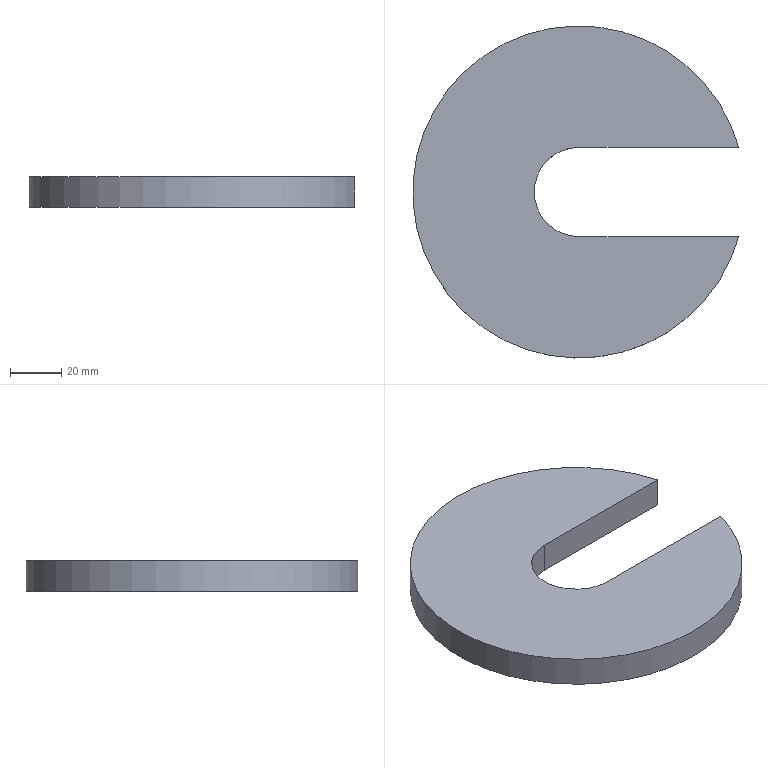Component | NX | QC_WASHER | 1 solid | 6 faces | box 127.6 x 130 x 12 mm | volume 126540 mm3 | plane 4 | cylinder 2 | commonest cylinder face diameters 35 x1 130 x1
STEP:
#1=CARTESIAN_POINT('',(0.,0.,0.));
#2=DIRECTION('',(0.,0.,1.));
#3=DIRECTION('',(1.,0.,0.));
#4=AXIS2_PLACEMENT_3D('',#1,#2,#3);
#5=CARTESIAN_POINT('',(62.6,-17.5,123.));
#6=VERTEX_POINT('',#5);
#7=CARTESIAN_POINT('',(0.,-17.5,123.));
#8=VERTEX_POINT('',#7);
#9=CARTESIAN_POINT('',(62.6,-17.5,123.));
#10=DIRECTION('',(-1.,-0.,0.));
#11=VECTOR('',#10,1.);
#12=LINE('',#9,#11);
#13=CARTESIAN_POINT('',(62.6,-17.5,135.));
#14=DIRECTION('',(0.,-1.,0.));
#15=DIRECTION('',(1.,0.,0.));
#16=AXIS2_PLACEMENT_3D('',#13,#14,#15);
#17=PLANE('',#16);
#18=CARTESIAN_POINT('',(0.,-12.));
#19=DIRECTION('',(-1.,0.));
#20=VECTOR('',#19,1.);
#21=LINE('',#18,#20);
#22=(GEOMETRIC_REPRESENTATION_CONTEXT(2)PARAMETRIC_REPRESENTATION_CONTEXT()REPRESENTATION_CONTEXT('',''));
#23=DEFINITIONAL_REPRESENTATION('',(#21),#22);
#24=PCURVE('',#17,#23);
#25=CARTESIAN_POINT('',(0.,0.,123.));
#26=DIRECTION('',(0.,0.,-1.));
#27=DIRECTION('',(0.,-1.,0.));
#28=AXIS2_PLACEMENT_3D('',#25,#26,#27);
#29=PLANE('',#28);
#30=CARTESIAN_POINT('',(17.5,-62.6));
#31=DIRECTION('',(0.,1.));
#32=VECTOR('',#31,1.);
#33=LINE('',#30,#32);
#34=(GEOMETRIC_REPRESENTATION_CONTEXT(2)PARAMETRIC_REPRESENTATION_CONTEXT()REPRESENTATION_CONTEXT('',''));
#35=DEFINITIONAL_REPRESENTATION('',(#33),#34);
#36=PCURVE('',#29,#35);
#37=SURFACE_CURVE('',#12,(#24,#36),.PCURVE_S1.);
#38=EDGE_CURVE('',#6,#8,#37,.T.);
#39=ORIENTED_EDGE('',*,*,#38,.T.);
#40=CARTESIAN_POINT('',(0.,-17.5,135.));
#41=VERTEX_POINT('',#40);
#42=CARTESIAN_POINT('',(0.,-17.5,135.));
#43=DIRECTION('',(0.,0.,-1.));
#44=VECTOR('',#43,1.);
#45=LINE('',#42,#44);
#46=CARTESIAN_POINT('',(-62.6,0.));
#47=DIRECTION('',(0.,-1.));
#48=VECTOR('',#47,1.);
#49=LINE('',#46,#48);
#50=(GEOMETRIC_REPRESENTATION_CONTEXT(2)PARAMETRIC_REPRESENTATION_CONTEXT()REPRESENTATION_CONTEXT('',''));
#51=DEFINITIONAL_REPRESENTATION('',(#49),#50);
#52=PCURVE('',#17,#51);
#53=CARTESIAN_POINT('',(0.,0.,135.));
#54=DIRECTION('',(0.,0.,-1.));
#55=DIRECTION('',(0.,-1.,0.));
#56=AXIS2_PLACEMENT_3D('',#53,#54,#55);
#57=CYLINDRICAL_SURFACE('',#56,17.5);
#58=CARTESIAN_POINT('',(0.,0.));
#59=DIRECTION('',(0.,1.));
#60=VECTOR('',#59,1.);
#61=LINE('',#58,#60);
#62=(GEOMETRIC_REPRESENTATION_CONTEXT(2)PARAMETRIC_REPRESENTATION_CONTEXT()REPRESENTATION_CONTEXT('',''));
#63=DEFINITIONAL_REPRESENTATION('',(#61),#62);
#64=PCURVE('',#57,#63);
#65=SURFACE_CURVE('',#45,(#52,#64),.PCURVE_S1.);
#66=EDGE_CURVE('',#41,#8,#65,.T.);
#67=ORIENTED_EDGE('',*,*,#66,.F.);
#68=CARTESIAN_POINT('',(62.6,-17.5,135.));
#69=VERTEX_POINT('',#68);
#70=CARTESIAN_POINT('',(62.6,-17.5,135.));
#71=DIRECTION('',(-1.,-0.,0.));
#72=VECTOR('',#71,1.);
#73=LINE('',#70,#72);
#74=CARTESIAN_POINT('',(0.,0.));
#75=DIRECTION('',(-1.,0.));
#76=VECTOR('',#75,1.);
#77=LINE('',#74,#76);
#78=(GEOMETRIC_REPRESENTATION_CONTEXT(2)PARAMETRIC_REPRESENTATION_CONTEXT()REPRESENTATION_CONTEXT('',''));
#79=DEFINITIONAL_REPRESENTATION('',(#77),#78);
#80=PCURVE('',#17,#79);
#81=CARTESIAN_POINT('',(0.,0.,135.));
#82=DIRECTION('',(0.,0.,-1.));
#83=DIRECTION('',(0.,-1.,0.));
#84=AXIS2_PLACEMENT_3D('',#81,#82,#83);
#85=PLANE('',#84);
#86=CARTESIAN_POINT('',(17.5,-62.6));
#87=DIRECTION('',(0.,1.));
#88=VECTOR('',#87,1.);
#89=LINE('',#86,#88);
#90=(GEOMETRIC_REPRESENTATION_CONTEXT(2)PARAMETRIC_REPRESENTATION_CONTEXT()REPRESENTATION_CONTEXT('',''));
#91=DEFINITIONAL_REPRESENTATION('',(#89),#90);
#92=PCURVE('',#85,#91);
#93=SURFACE_CURVE('',#73,(#80,#92),.PCURVE_S1.);
#94=EDGE_CURVE('',#69,#41,#93,.T.);
#95=ORIENTED_EDGE('',*,*,#94,.F.);
#96=CARTESIAN_POINT('',(62.6,-17.5,135.));
#97=DIRECTION('',(0.,0.,-1.));
#98=VECTOR('',#97,1.);
#99=LINE('',#96,#98);
#100=CARTESIAN_POINT('',(0.,0.));
#101=DIRECTION('',(0.,-1.));
#102=VECTOR('',#101,1.);
#103=LINE('',#100,#102);
#104=(GEOMETRIC_REPRESENTATION_CONTEXT(2)PARAMETRIC_REPRESENTATION_CONTEXT()REPRESENTATION_CONTEXT('',''));
#105=DEFINITIONAL_REPRESENTATION('',(#103),#104);
#106=PCURVE('',#17,#105);
#107=CARTESIAN_POINT('',(0.,0.,135.));
#108=DIRECTION('',(0.,0.,-1.));
#109=DIRECTION('',(0.,-1.,0.));
#110=AXIS2_PLACEMENT_3D('',#107,#108,#109);
#111=CYLINDRICAL_SURFACE('',#110,65.);
#112=CARTESIAN_POINT('',(-1.298,0.));
#113=DIRECTION('',(0.,1.));
#114=VECTOR('',#113,1.);
#115=LINE('',#112,#114);
#116=(GEOMETRIC_REPRESENTATION_CONTEXT(2)PARAMETRIC_REPRESENTATION_CONTEXT()REPRESENTATION_CONTEXT('',''));
#117=DEFINITIONAL_REPRESENTATION('',(#115),#116);
#118=PCURVE('',#111,#117);
#119=SURFACE_CURVE('',#99,(#106,#118),.PCURVE_S1.);
#120=EDGE_CURVE('',#69,#6,#119,.T.);
#121=ORIENTED_EDGE('',*,*,#120,.T.);
#122=EDGE_LOOP('',(#39,#67,#95,#121));
#123=FACE_BOUND('',#122,.T.);
#124=ADVANCED_FACE('',(#123),#17,.F.);
#125=ORIENTED_EDGE('',*,*,#66,.F.);
#126=CARTESIAN_POINT('',(-0.,17.5,135.));
#127=VERTEX_POINT('',#126);
#128=CARTESIAN_POINT('',(0.,0.,135.));
#129=DIRECTION('',(0.,0.,-1.));
#130=DIRECTION('',(-0.,1.,0.));
#131=AXIS2_PLACEMENT_3D('',#128,#129,#130);
#132=CIRCLE('',#131,17.5);
#133=CARTESIAN_POINT('',(-3.142,0.));
#134=DIRECTION('',(1.,0.));
#135=VECTOR('',#134,1.);
#136=LINE('',#133,#135);
#137=(GEOMETRIC_REPRESENTATION_CONTEXT(2)PARAMETRIC_REPRESENTATION_CONTEXT()REPRESENTATION_CONTEXT('',''));
#138=DEFINITIONAL_REPRESENTATION('',(#136),#137);
#139=PCURVE('',#57,#138);
#140=CARTESIAN_POINT('',(0.,0.));
#141=DIRECTION('',(-1.,0.));
#142=AXIS2_PLACEMENT_2D('',#140,#141);
#143=CIRCLE('',#142,17.5);
#144=(GEOMETRIC_REPRESENTATION_CONTEXT(2)PARAMETRIC_REPRESENTATION_CONTEXT()REPRESENTATION_CONTEXT('',''));
#145=DEFINITIONAL_REPRESENTATION('',(#143),#144);
#146=PCURVE('',#85,#145);
#147=SURFACE_CURVE('',#132,(#139,#146),.PCURVE_S1.);
#148=EDGE_CURVE('',#41,#127,#147,.T.);
#149=ORIENTED_EDGE('',*,*,#148,.T.);
#150=CARTESIAN_POINT('',(-0.,17.5,123.));
#151=VERTEX_POINT('',#150);
#152=CARTESIAN_POINT('',(-0.,17.5,135.));
#153=DIRECTION('',(0.,0.,-1.));
#154=VECTOR('',#153,1.);
#155=LINE('',#152,#154);
#156=CARTESIAN_POINT('',(3.142,0.));
#157=DIRECTION('',(0.,1.));
#158=VECTOR('',#157,1.);
#159=LINE('',#156,#158);
#160=(GEOMETRIC_REPRESENTATION_CONTEXT(2)PARAMETRIC_REPRESENTATION_CONTEXT()REPRESENTATION_CONTEXT('',''));
#161=DEFINITIONAL_REPRESENTATION('',(#159),#160);
#162=PCURVE('',#57,#161);
#163=CARTESIAN_POINT('',(0.,17.5,135.));
#164=DIRECTION('',(-0.,1.,0.));
#165=DIRECTION('',(-1.,-0.,0.));
#166=AXIS2_PLACEMENT_3D('',#163,#164,#165);
#167=PLANE('',#166);
#168=CARTESIAN_POINT('',(0.,0.));
#169=DIRECTION('',(0.,-1.));
#170=VECTOR('',#169,1.);
#171=LINE('',#168,#170);
#172=(GEOMETRIC_REPRESENTATION_CONTEXT(2)PARAMETRIC_REPRESENTATION_CONTEXT()REPRESENTATION_CONTEXT('',''));
#173=DEFINITIONAL_REPRESENTATION('',(#171),#172);
#174=PCURVE('',#167,#173);
#175=SURFACE_CURVE('',#155,(#162,#174),.PCURVE_S1.);
#176=EDGE_CURVE('',#127,#151,#175,.T.);
#177=ORIENTED_EDGE('',*,*,#176,.T.);
#178=CARTESIAN_POINT('',(0.,0.,123.));
#179=DIRECTION('',(0.,0.,-1.));
#180=DIRECTION('',(-0.,1.,0.));
#181=AXIS2_PLACEMENT_3D('',#178,#179,#180);
#182=CIRCLE('',#181,17.5);
#183=CARTESIAN_POINT('',(-3.142,12.));
#184=DIRECTION('',(1.,0.));
#185=VECTOR('',#184,1.);
#186=LINE('',#183,#185);
#187=(GEOMETRIC_REPRESENTATION_CONTEXT(2)PARAMETRIC_REPRESENTATION_CONTEXT()REPRESENTATION_CONTEXT('',''));
#188=DEFINITIONAL_REPRESENTATION('',(#186),#187);
#189=PCURVE('',#57,#188);
#190=CARTESIAN_POINT('',(0.,0.));
#191=DIRECTION('',(-1.,0.));
#192=AXIS2_PLACEMENT_2D('',#190,#191);
#193=CIRCLE('',#192,17.5);
#194=(GEOMETRIC_REPRESENTATION_CONTEXT(2)PARAMETRIC_REPRESENTATION_CONTEXT()REPRESENTATION_CONTEXT('',''));
#195=DEFINITIONAL_REPRESENTATION('',(#193),#194);
#196=PCURVE('',#29,#195);
#197=SURFACE_CURVE('',#182,(#189,#196),.PCURVE_S1.);
#198=EDGE_CURVE('',#8,#151,#197,.T.);
#199=ORIENTED_EDGE('',*,*,#198,.F.);
#200=EDGE_LOOP('',(#125,#149,#177,#199));
#201=FACE_BOUND('',#200,.F.);
#202=ADVANCED_FACE('',(#201),#57,.F.);
#203=CARTESIAN_POINT('',(62.6,17.5,123.));
#204=VERTEX_POINT('',#203);
#205=CARTESIAN_POINT('',(0.,17.5,123.));
#206=DIRECTION('',(1.,0.,0.));
#207=VECTOR('',#206,1.);
#208=LINE('',#205,#207);
#209=CARTESIAN_POINT('',(0.,-12.));
#210=DIRECTION('',(-1.,0.));
#211=VECTOR('',#210,1.);
#212=LINE('',#209,#211);
#213=(GEOMETRIC_REPRESENTATION_CONTEXT(2)PARAMETRIC_REPRESENTATION_CONTEXT()REPRESENTATION_CONTEXT('',''));
#214=DEFINITIONAL_REPRESENTATION('',(#212),#213);
#215=PCURVE('',#167,#214);
#216=CARTESIAN_POINT('',(-17.5,-0.));
#217=DIRECTION('',(-0.,-1.));
#218=VECTOR('',#217,1.);
#219=LINE('',#216,#218);
#220=(GEOMETRIC_REPRESENTATION_CONTEXT(2)PARAMETRIC_REPRESENTATION_CONTEXT()REPRESENTATION_CONTEXT('',''));
#221=DEFINITIONAL_REPRESENTATION('',(#219),#220);
#222=PCURVE('',#29,#221);
#223=SURFACE_CURVE('',#208,(#215,#222),.PCURVE_S1.);
#224=EDGE_CURVE('',#151,#204,#223,.T.);
#225=ORIENTED_EDGE('',*,*,#224,.T.);
#226=CARTESIAN_POINT('',(62.6,17.5,135.));
#227=VERTEX_POINT('',#226);
#228=CARTESIAN_POINT('',(62.6,17.5,135.));
#229=DIRECTION('',(0.,0.,-1.));
#230=VECTOR('',#229,1.);
#231=LINE('',#228,#230);
#232=CARTESIAN_POINT('',(-62.6,0.));
#233=DIRECTION('',(0.,-1.));
#234=VECTOR('',#233,1.);
#235=LINE('',#232,#234);
#236=(GEOMETRIC_REPRESENTATION_CONTEXT(2)PARAMETRIC_REPRESENTATION_CONTEXT()REPRESENTATION_CONTEXT('',''));
#237=DEFINITIONAL_REPRESENTATION('',(#235),#236);
#238=PCURVE('',#167,#237);
#239=CARTESIAN_POINT('',(4.44,0.));
#240=DIRECTION('',(0.,1.));
#241=VECTOR('',#240,1.);
#242=LINE('',#239,#241);
#243=(GEOMETRIC_REPRESENTATION_CONTEXT(2)PARAMETRIC_REPRESENTATION_CONTEXT()REPRESENTATION_CONTEXT('',''));
#244=DEFINITIONAL_REPRESENTATION('',(#242),#243);
#245=PCURVE('',#111,#244);
#246=SURFACE_CURVE('',#231,(#238,#245),.PCURVE_S1.);
#247=EDGE_CURVE('',#227,#204,#246,.T.);
#248=ORIENTED_EDGE('',*,*,#247,.F.);
#249=CARTESIAN_POINT('',(0.,17.5,135.));
#250=DIRECTION('',(1.,0.,0.));
#251=VECTOR('',#250,1.);
#252=LINE('',#249,#251);
#253=CARTESIAN_POINT('',(0.,0.));
#254=DIRECTION('',(-1.,0.));
#255=VECTOR('',#254,1.);
#256=LINE('',#253,#255);
#257=(GEOMETRIC_REPRESENTATION_CONTEXT(2)PARAMETRIC_REPRESENTATION_CONTEXT()REPRESENTATION_CONTEXT('',''));
#258=DEFINITIONAL_REPRESENTATION('',(#256),#257);
#259=PCURVE('',#167,#258);
#260=CARTESIAN_POINT('',(-17.5,-0.));
#261=DIRECTION('',(-0.,-1.));
#262=VECTOR('',#261,1.);
#263=LINE('',#260,#262);
#264=(GEOMETRIC_REPRESENTATION_CONTEXT(2)PARAMETRIC_REPRESENTATION_CONTEXT()REPRESENTATION_CONTEXT('',''));
#265=DEFINITIONAL_REPRESENTATION('',(#263),#264);
#266=PCURVE('',#85,#265);
#267=SURFACE_CURVE('',#252,(#259,#266),.PCURVE_S1.);
#268=EDGE_CURVE('',#127,#227,#267,.T.);
#269=ORIENTED_EDGE('',*,*,#268,.F.);
#270=ORIENTED_EDGE('',*,*,#176,.T.);
#271=EDGE_LOOP('',(#225,#248,#269,#270));
#272=FACE_BOUND('',#271,.T.);
#273=ADVANCED_FACE('',(#272),#167,.F.);
#274=CARTESIAN_POINT('',(0.,0.,123.));
#275=DIRECTION('',(0.,0.,1.));
#276=DIRECTION('',(0.,1.,0.));
#277=AXIS2_PLACEMENT_3D('',#274,#275,#276);
#278=CIRCLE('',#277,65.);
#279=CARTESIAN_POINT('',(9.425,12.));
#280=DIRECTION('',(-1.,0.));
#281=VECTOR('',#280,1.);
#282=LINE('',#279,#281);
#283=(GEOMETRIC_REPRESENTATION_CONTEXT(2)PARAMETRIC_REPRESENTATION_CONTEXT()REPRESENTATION_CONTEXT('',''));
#284=DEFINITIONAL_REPRESENTATION('',(#282),#283);
#285=PCURVE('',#111,#284);
#286=CARTESIAN_POINT('',(-65.,0.));
#287=CARTESIAN_POINT('',(-65.,112.583));
#288=CARTESIAN_POINT('',(32.5,56.292));
#289=CARTESIAN_POINT('',(130.,0.));
#290=CARTESIAN_POINT('',(32.5,-56.292));
#291=CARTESIAN_POINT('',(-65.,-112.583));
#292=CARTESIAN_POINT('',(-65.,0.));
#293=(BOUNDED_CURVE()B_SPLINE_CURVE(2,(#286,#287,#288,#289,#290,#291,#292),.UNSPECIFIED.,.T.,.F.)B_SPLINE_CURVE_WITH_KNOTS((1,2,2,2,2,1),(-2.094,0.,2.094,4.189,6.283,8.378),.UNSPECIFIED.)CURVE()GEOMETRIC_REPRESENTATION_ITEM()RATIONAL_B_SPLINE_CURVE((1.,0.5,1.,0.5,1.,0.5,1.))REPRESENTATION_ITEM(''));
#294=(GEOMETRIC_REPRESENTATION_CONTEXT(2)PARAMETRIC_REPRESENTATION_CONTEXT()REPRESENTATION_CONTEXT('',''));
#295=DEFINITIONAL_REPRESENTATION('',(#293),#294);
#296=PCURVE('',#29,#295);
#297=SURFACE_CURVE('',#278,(#285,#296),.PCURVE_S1.);
#298=EDGE_CURVE('',#204,#6,#297,.T.);
#299=ORIENTED_EDGE('',*,*,#298,.T.);
#300=ORIENTED_EDGE('',*,*,#120,.F.);
#301=CARTESIAN_POINT('',(0.,0.,135.));
#302=DIRECTION('',(0.,0.,1.));
#303=DIRECTION('',(0.,1.,0.));
#304=AXIS2_PLACEMENT_3D('',#301,#302,#303);
#305=CIRCLE('',#304,65.);
#306=CARTESIAN_POINT('',(9.425,0.));
#307=DIRECTION('',(-1.,0.));
#308=VECTOR('',#307,1.);
#309=LINE('',#306,#308);
#310=(GEOMETRIC_REPRESENTATION_CONTEXT(2)PARAMETRIC_REPRESENTATION_CONTEXT()REPRESENTATION_CONTEXT('',''));
#311=DEFINITIONAL_REPRESENTATION('',(#309),#310);
#312=PCURVE('',#111,#311);
#313=CARTESIAN_POINT('',(-65.,0.));
#314=CARTESIAN_POINT('',(-65.,112.583));
#315=CARTESIAN_POINT('',(32.5,56.292));
#316=CARTESIAN_POINT('',(130.,0.));
#317=CARTESIAN_POINT('',(32.5,-56.292));
#318=CARTESIAN_POINT('',(-65.,-112.583));
#319=CARTESIAN_POINT('',(-65.,0.));
#320=(BOUNDED_CURVE()B_SPLINE_CURVE(2,(#313,#314,#315,#316,#317,#318,#319),.UNSPECIFIED.,.T.,.F.)B_SPLINE_CURVE_WITH_KNOTS((1,2,2,2,2,1),(-2.094,0.,2.094,4.189,6.283,8.378),.UNSPECIFIED.)CURVE()GEOMETRIC_REPRESENTATION_ITEM()RATIONAL_B_SPLINE_CURVE((1.,0.5,1.,0.5,1.,0.5,1.))REPRESENTATION_ITEM(''));
#321=(GEOMETRIC_REPRESENTATION_CONTEXT(2)PARAMETRIC_REPRESENTATION_CONTEXT()REPRESENTATION_CONTEXT('',''));
#322=DEFINITIONAL_REPRESENTATION('',(#320),#321);
#323=PCURVE('',#85,#322);
#324=SURFACE_CURVE('',#305,(#312,#323),.PCURVE_S1.);
#325=EDGE_CURVE('',#227,#69,#324,.T.);
#326=ORIENTED_EDGE('',*,*,#325,.F.);
#327=ORIENTED_EDGE('',*,*,#247,.T.);
#328=EDGE_LOOP('',(#299,#300,#326,#327));
#329=FACE_BOUND('',#328,.T.);
#330=ADVANCED_FACE('',(#329),#111,.T.);
#331=ORIENTED_EDGE('',*,*,#94,.T.);
#332=ORIENTED_EDGE('',*,*,#148,.T.);
#333=ORIENTED_EDGE('',*,*,#268,.T.);
#334=ORIENTED_EDGE('',*,*,#325,.T.);
#335=EDGE_LOOP('',(#331,#332,#333,#334));
#336=FACE_BOUND('',#335,.T.);
#337=ADVANCED_FACE('',(#336),#85,.F.);
#338=ORIENTED_EDGE('',*,*,#38,.F.);
#339=ORIENTED_EDGE('',*,*,#298,.F.);
#340=ORIENTED_EDGE('',*,*,#224,.F.);
#341=ORIENTED_EDGE('',*,*,#198,.F.);
#342=EDGE_LOOP('',(#338,#339,#340,#341));
#343=FACE_BOUND('',#342,.T.);
#344=ADVANCED_FACE('',(#343),#29,.T.);
#345=CLOSED_SHELL('',(#124,#202,#273,#330,#337,#344));
#346=MANIFOLD_SOLID_BREP('',#345);
#347=(LENGTH_UNIT()NAMED_UNIT(*)SI_UNIT(.MILLI.,.METRE.));
#348=UNCERTAINTY_MEASURE_WITH_UNIT(LENGTH_MEASURE(0.0000001),#347,'','');
#349=(NAMED_UNIT(*)PLANE_ANGLE_UNIT()SI_UNIT($,.RADIAN.));
#350=(NAMED_UNIT(*)SI_UNIT($,.STERADIAN.)SOLID_ANGLE_UNIT());
#351=(GEOMETRIC_REPRESENTATION_CONTEXT(3)GLOBAL_UNCERTAINTY_ASSIGNED_CONTEXT((#348))GLOBAL_UNIT_ASSIGNED_CONTEXT((#347,#349,#350))REPRESENTATION_CONTEXT('',''));
#352=ADVANCED_BREP_SHAPE_REPRESENTATION('',(#4,#346),#351);